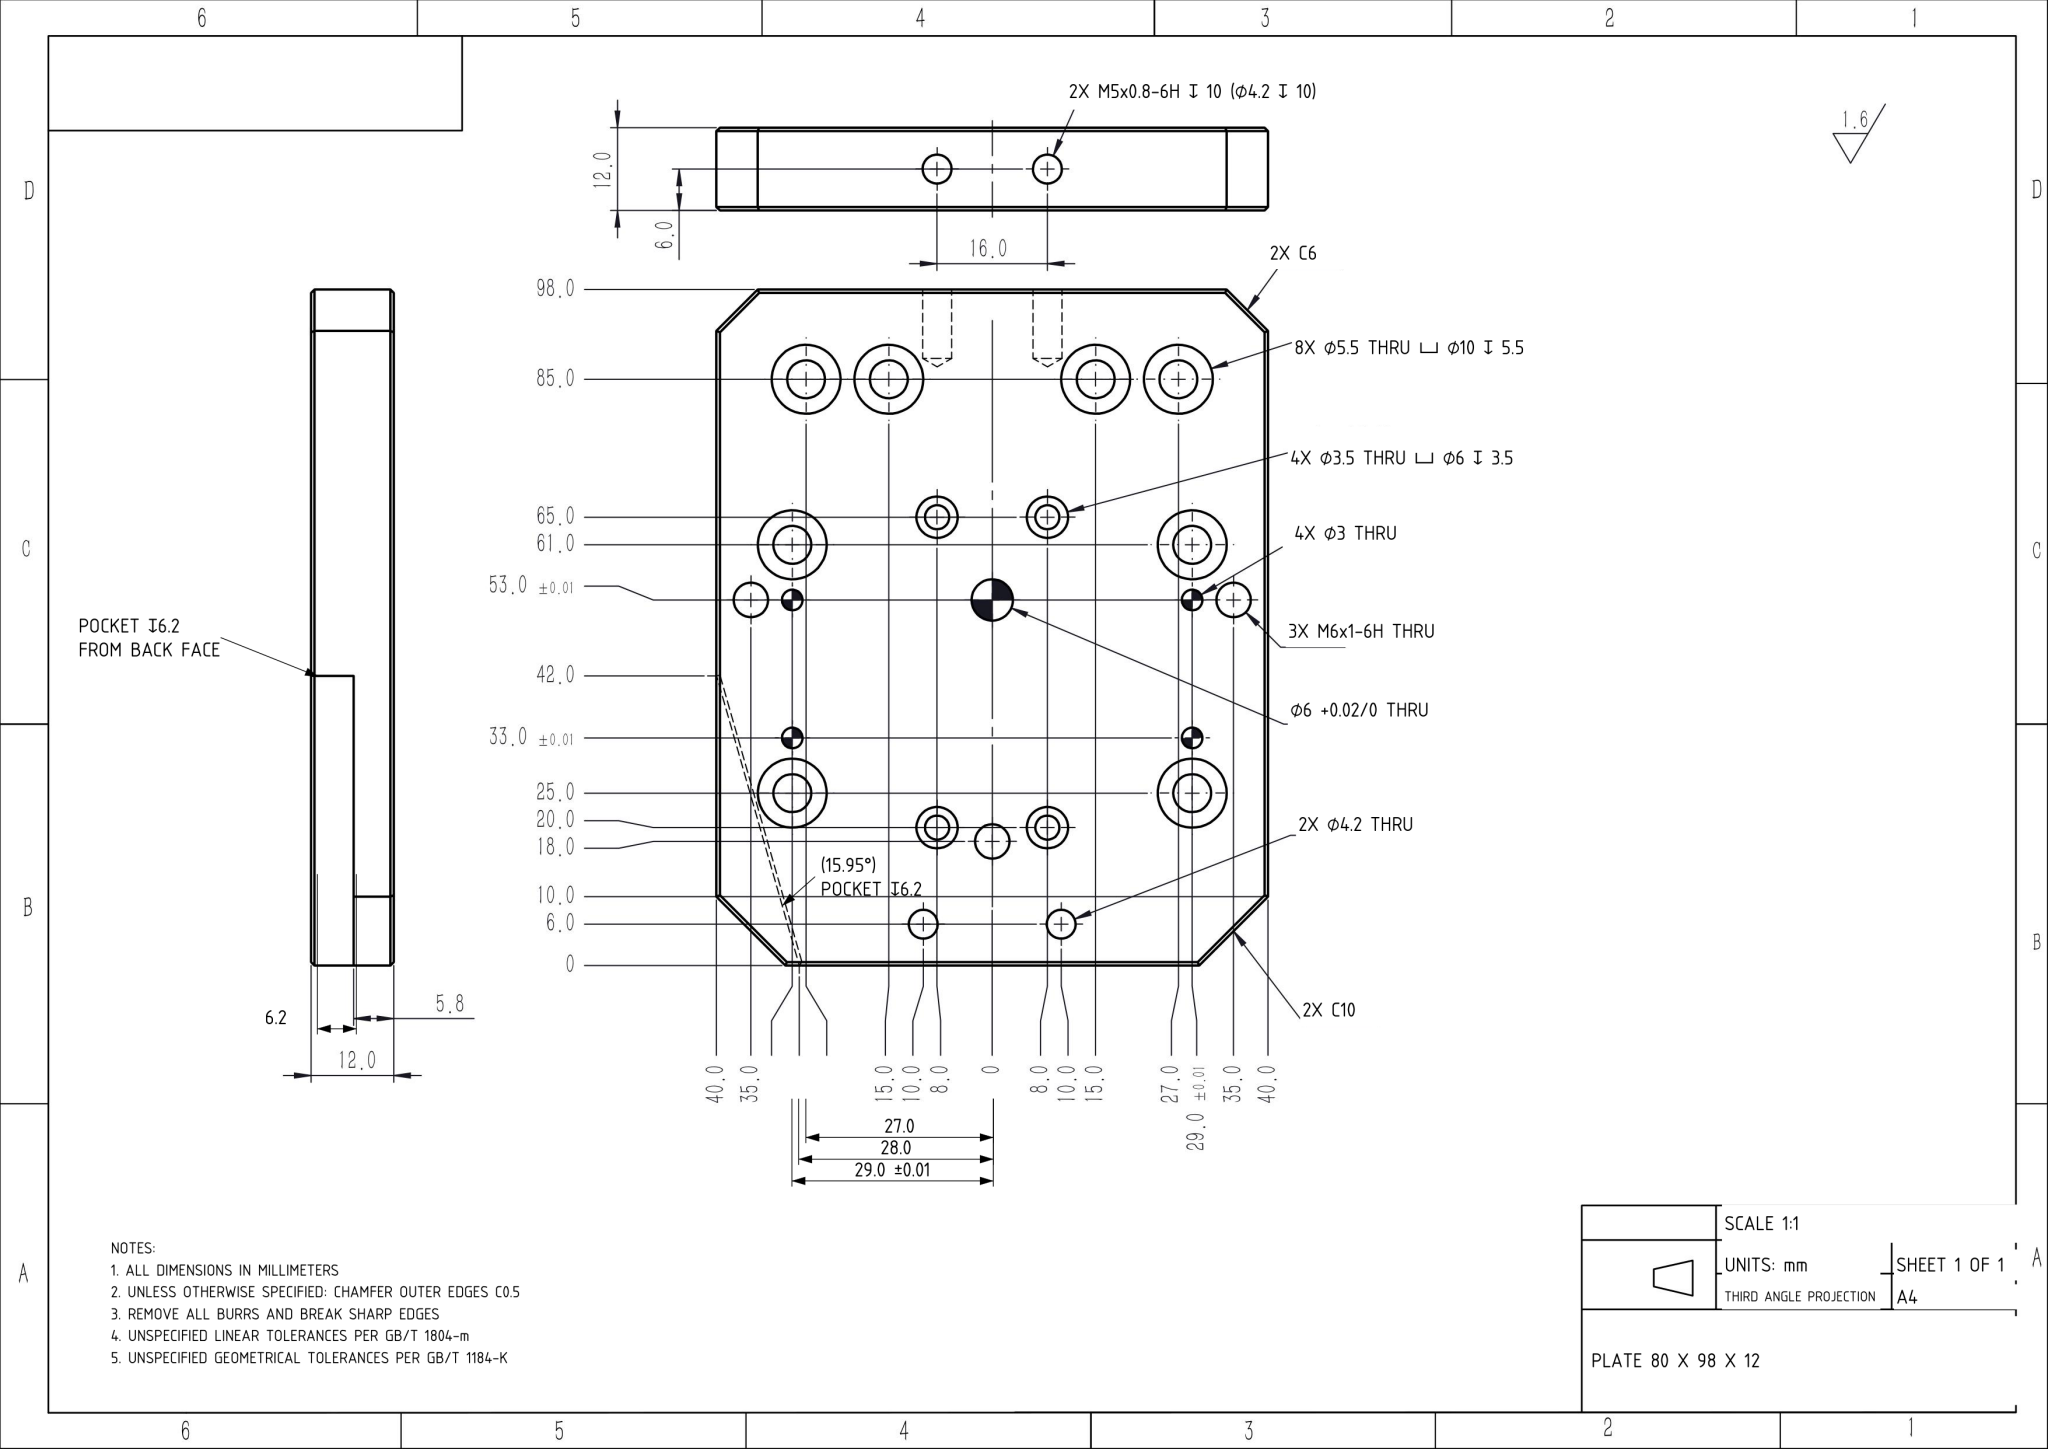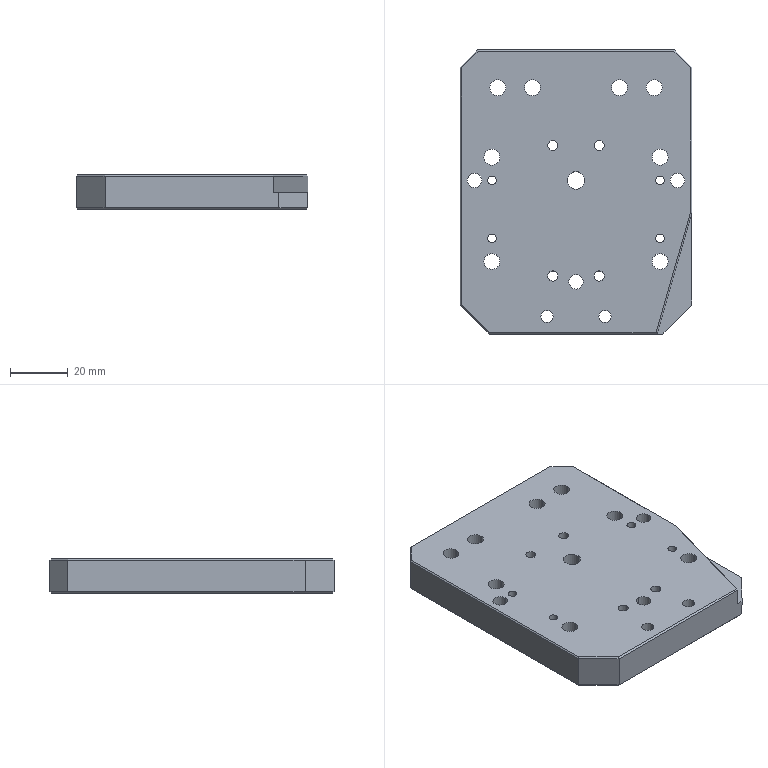Part | NX | mm | 1 solid | 116 faces | box 80 x 98 x 12 mm | volume 83692 mm3 | cylinder 72 | plane 40 | cone 4 | commonest cylinder face diameters 10 x16 5.5 x16 6 x10 3 x8 4.2 x8 3.5 x8 5 x6